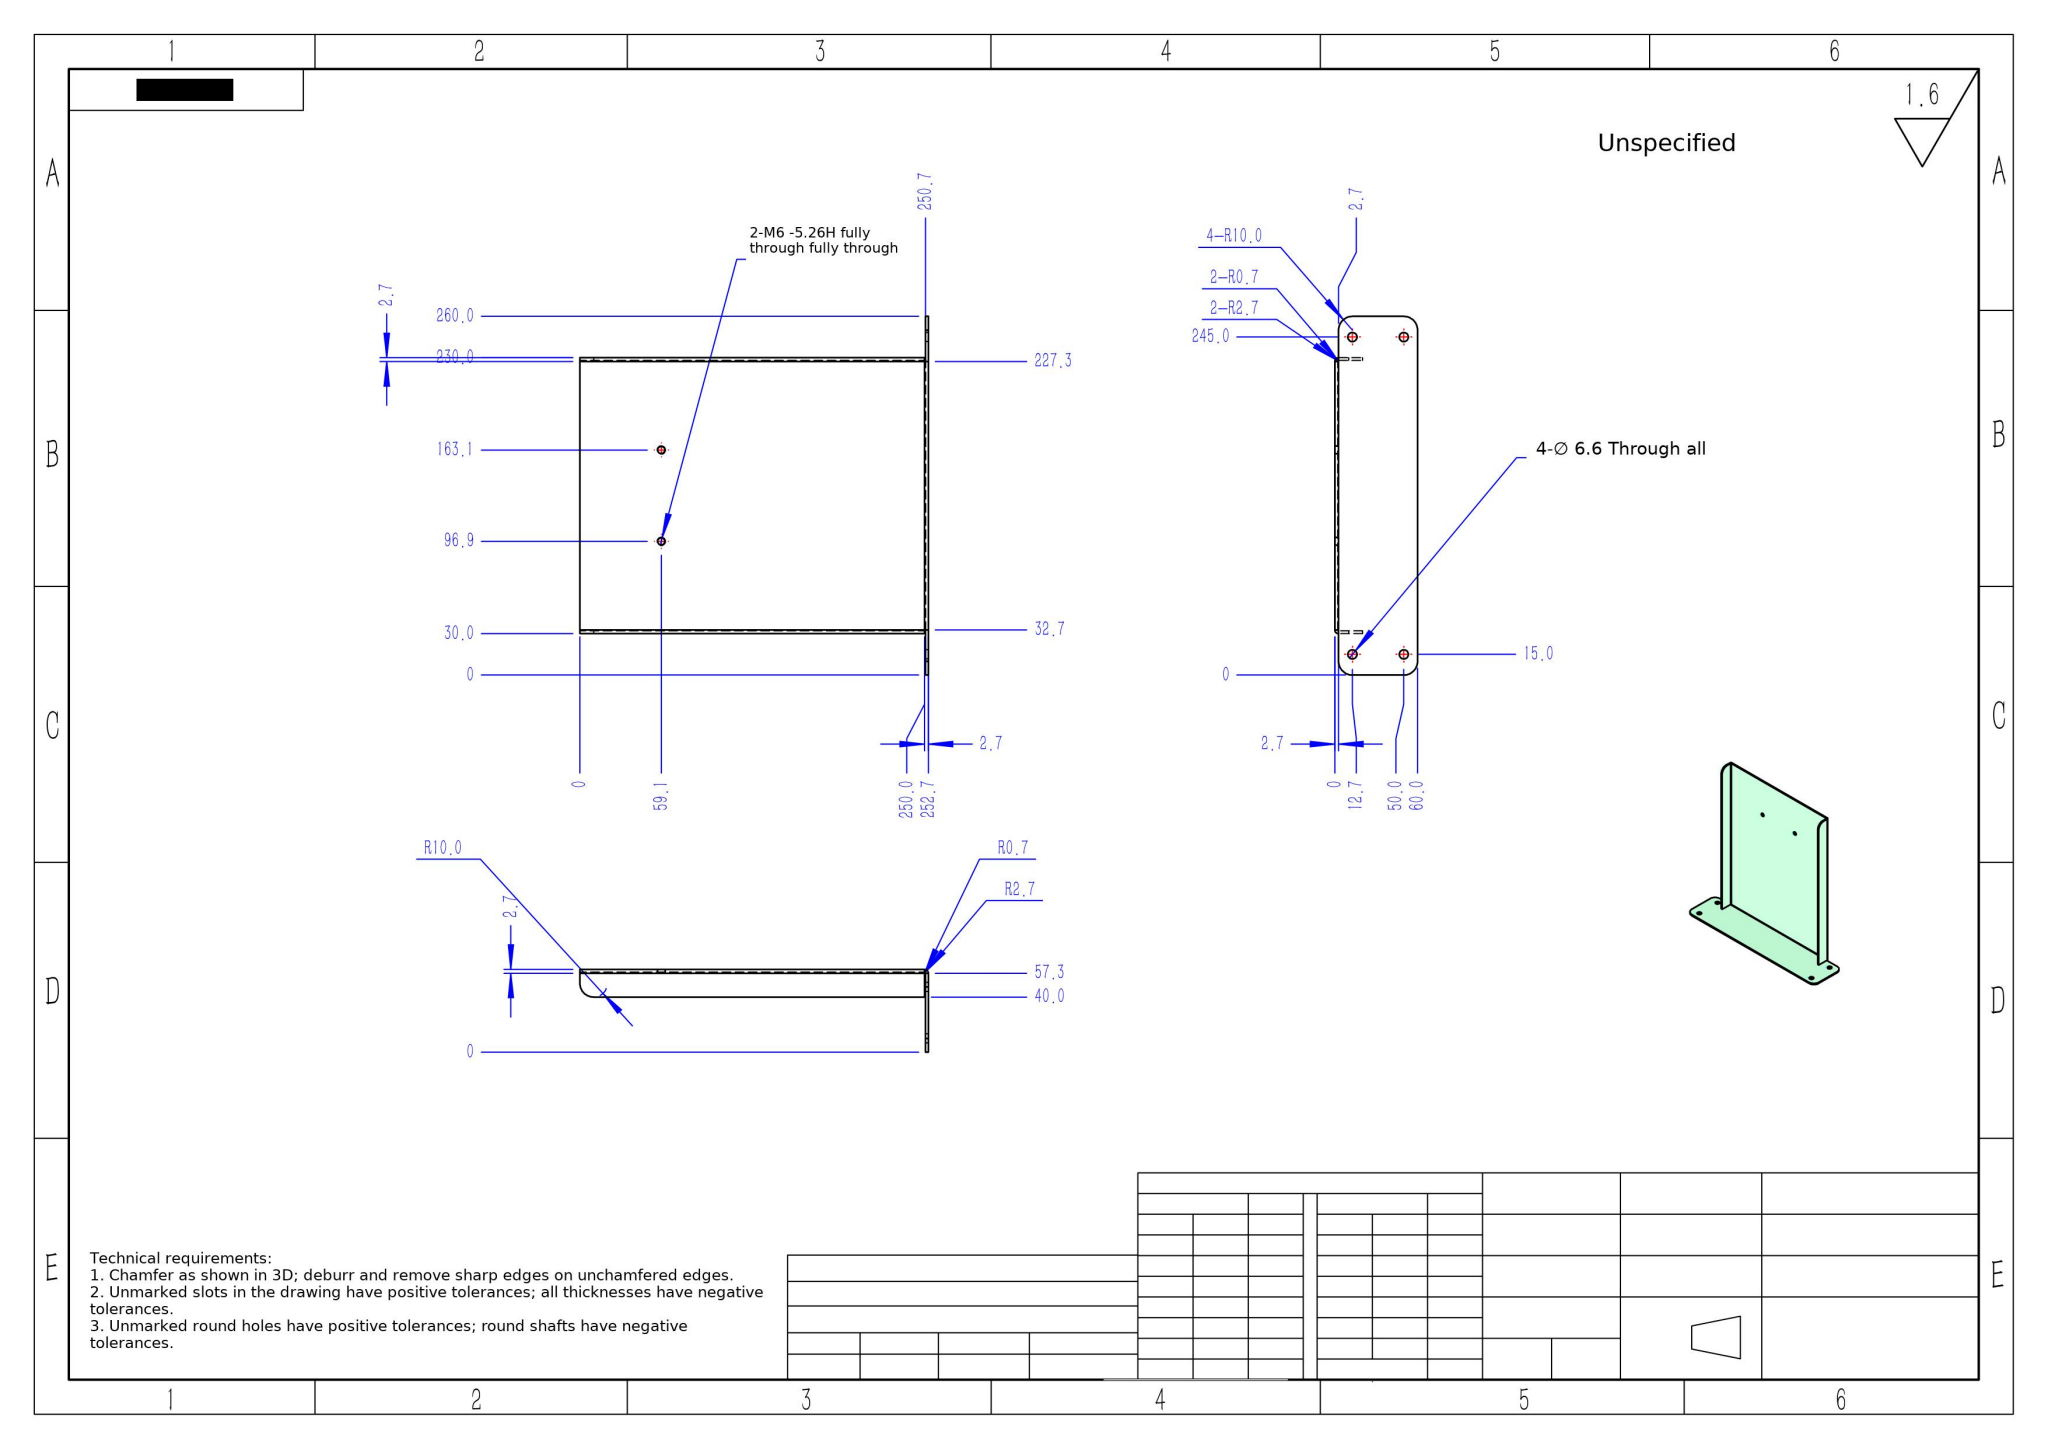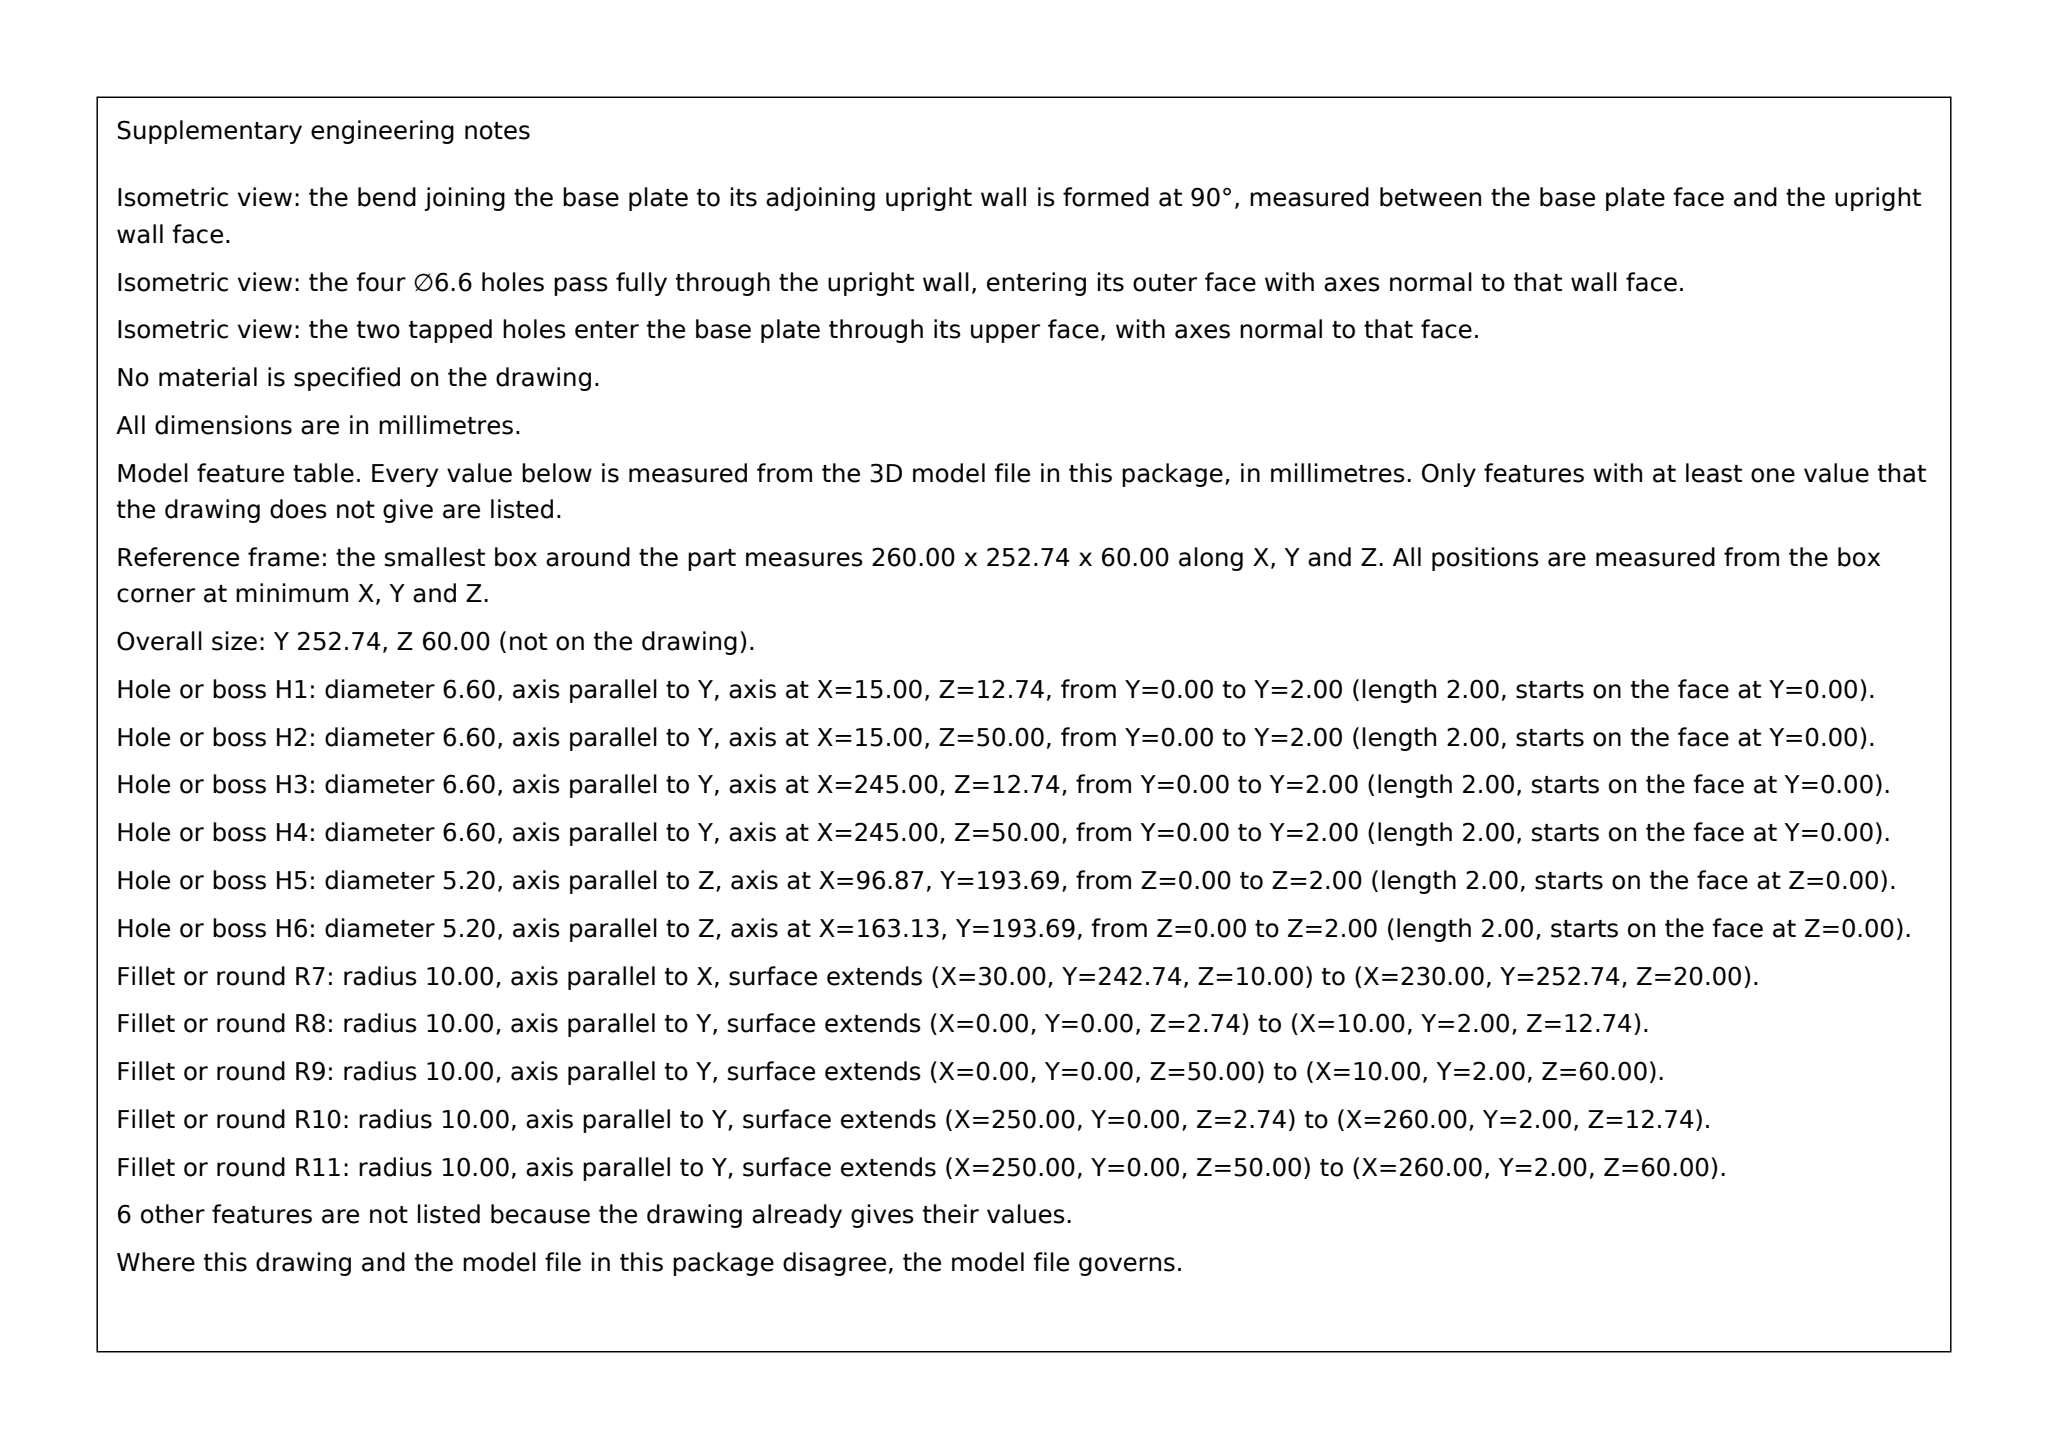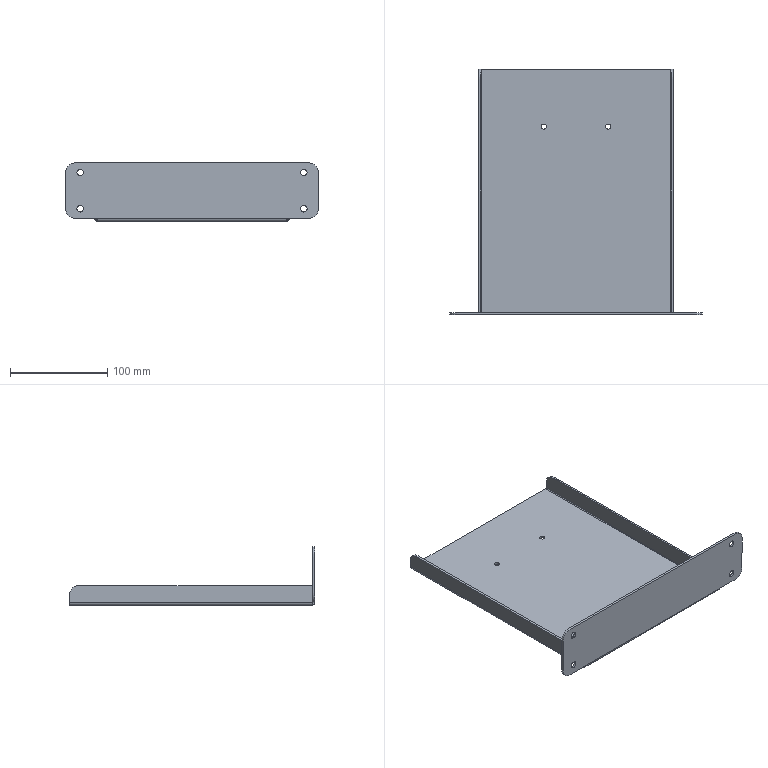Part | SolidWorks | mm | 1 solid | 50 faces | box 260 x 252.74 x 60 mm | volume 147477 mm3 | plane 26 | cylinder 24 | commonest cylinder face diameters 6.6 x8 20 x6 5.2 x4 5.473 x3 1.473 x3